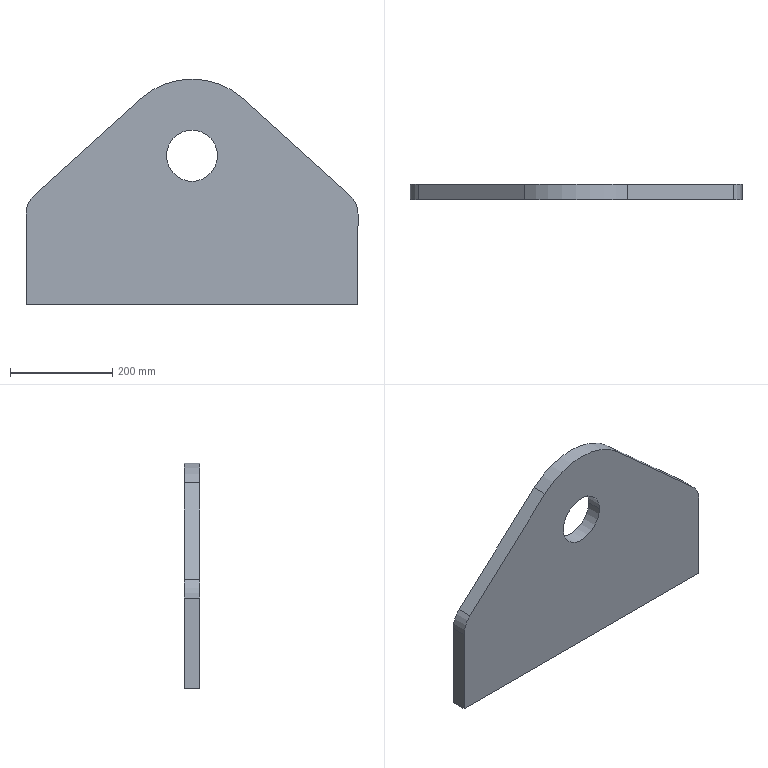Component | SolidWorks | Support1-1 | 1 solid | 12 faces | box 650 x 30 x 442 mm | volume 6416148 mm3 | plane 7 | cylinder 5 | commonest cylinder face diameters 100 x4 300 x1 | material Plain Carbon Steel
STEP:
#1=COLOUR_RGB('',0.7922,0.8196,0.9333);
#2=FILL_AREA_STYLE_COLOUR('',#1);
#3=FILL_AREA_STYLE('',(#2));
#4=SURFACE_STYLE_FILL_AREA(#3);
#5=SURFACE_SIDE_STYLE('',(#4));
#6=SURFACE_STYLE_USAGE(.BOTH.,#5);
#7=PRESENTATION_STYLE_ASSIGNMENT((#6));
#8=CARTESIAN_POINT('',(47.267,41.982,72.956));
#9=VERTEX_POINT('',#8);
#10=CARTESIAN_POINT('',(51.204,41.982,72.956));
#11=VERTEX_POINT('',#10);
#12=CARTESIAN_POINT('',(49.235,41.982,72.956));
#13=DIRECTION('',(0.,1.,0.));
#14=DIRECTION('',(1.,0.,0.));
#15=AXIS2_PLACEMENT_3D('',#12,#13,#14);
#16=CIRCLE('',#15,1.969);
#17=EDGE_CURVE('',#9,#11,#16,.T.);
#18=ORIENTED_EDGE('',*,*,#17,.F.);
#19=CARTESIAN_POINT('',(47.267,43.163,72.956));
#20=VERTEX_POINT('',#19);
#21=CARTESIAN_POINT('',(47.267,41.982,72.956));
#22=DIRECTION('',(0.,1.,0.));
#23=VECTOR('',#22,39.37);
#24=LINE('',#21,#23);
#25=EDGE_CURVE('',#9,#20,#24,.T.);
#26=ORIENTED_EDGE('',*,*,#25,.T.);
#27=CARTESIAN_POINT('',(51.204,43.163,72.956));
#28=VERTEX_POINT('',#27);
#29=CARTESIAN_POINT('',(49.235,43.163,72.956));
#30=DIRECTION('',(0.,1.,0.));
#31=DIRECTION('',(1.,0.,0.));
#32=AXIS2_PLACEMENT_3D('',#29,#30,#31);
#33=CIRCLE('',#32,1.969);
#34=EDGE_CURVE('',#20,#28,#33,.T.);
#35=ORIENTED_EDGE('',*,*,#34,.T.);
#36=CARTESIAN_POINT('',(51.204,41.982,72.956));
#37=DIRECTION('',(0.,1.,0.));
#38=VECTOR('',#37,39.37);
#39=LINE('',#36,#38);
#40=EDGE_CURVE('',#11,#28,#39,.T.);
#41=ORIENTED_EDGE('',*,*,#40,.F.);
#42=EDGE_LOOP('',(#18,#26,#35,#41));
#43=FACE_OUTER_BOUND('',#42,.T.);
#44=CARTESIAN_POINT('',(49.235,41.982,72.956));
#45=DIRECTION('',(0.,1.,0.));
#46=DIRECTION('',(1.,0.,0.));
#47=AXIS2_PLACEMENT_3D('',#44,#45,#46);
#48=CYLINDRICAL_SURFACE('',#47,1.969);
#49=ADVANCED_FACE('',(#43),#48,.F.);
#50=CARTESIAN_POINT('',(36.44,43.163,61.46));
#51=VERTEX_POINT('',#50);
#52=CARTESIAN_POINT('',(36.44,43.163,68.461));
#53=VERTEX_POINT('',#52);
#54=CARTESIAN_POINT('',(36.44,43.163,61.46));
#55=DIRECTION('',(0.,-0.,1.));
#56=VECTOR('',#55,39.37);
#57=LINE('',#54,#56);
#58=EDGE_CURVE('',#51,#53,#57,.T.);
#59=ORIENTED_EDGE('',*,*,#58,.F.);
#60=CARTESIAN_POINT('',(36.44,41.982,61.46));
#61=VERTEX_POINT('',#60);
#62=CARTESIAN_POINT('',(36.44,41.982,61.46));
#63=DIRECTION('',(0.,1.,0.));
#64=VECTOR('',#63,39.37);
#65=LINE('',#62,#64);
#66=EDGE_CURVE('',#61,#51,#65,.T.);
#67=ORIENTED_EDGE('',*,*,#66,.F.);
#68=CARTESIAN_POINT('',(36.44,41.982,68.461));
#69=VERTEX_POINT('',#68);
#70=CARTESIAN_POINT('',(36.44,41.982,61.46));
#71=DIRECTION('',(0.,-0.,1.));
#72=VECTOR('',#71,39.37);
#73=LINE('',#70,#72);
#74=EDGE_CURVE('',#61,#69,#73,.T.);
#75=ORIENTED_EDGE('',*,*,#74,.T.);
#76=CARTESIAN_POINT('',(36.44,41.982,68.461));
#77=DIRECTION('',(0.,1.,0.));
#78=VECTOR('',#77,39.37);
#79=LINE('',#76,#78);
#80=EDGE_CURVE('',#69,#53,#79,.T.);
#81=ORIENTED_EDGE('',*,*,#80,.T.);
#82=EDGE_LOOP('',(#59,#67,#75,#81));
#83=FACE_OUTER_BOUND('',#82,.T.);
#84=CARTESIAN_POINT('',(36.44,41.982,61.46));
#85=DIRECTION('',(-1.,0.,0.));
#86=DIRECTION('',(0.,1.,0.));
#87=AXIS2_PLACEMENT_3D('',#84,#85,#86);
#88=PLANE('',#87);
#89=ADVANCED_FACE('',(#83),#88,.T.);
#90=CARTESIAN_POINT('',(62.031,43.163,61.46));
#91=VERTEX_POINT('',#90);
#92=CARTESIAN_POINT('',(36.44,43.163,61.46));
#93=DIRECTION('',(-1.,0.,0.));
#94=VECTOR('',#93,39.37);
#95=LINE('',#92,#94);
#96=EDGE_CURVE('',#91,#51,#95,.T.);
#97=ORIENTED_EDGE('',*,*,#96,.F.);
#98=CARTESIAN_POINT('',(62.031,41.982,61.46));
#99=VERTEX_POINT('',#98);
#100=CARTESIAN_POINT('',(62.031,41.982,61.46));
#101=DIRECTION('',(0.,1.,0.));
#102=VECTOR('',#101,39.37);
#103=LINE('',#100,#102);
#104=EDGE_CURVE('',#99,#91,#103,.T.);
#105=ORIENTED_EDGE('',*,*,#104,.F.);
#106=CARTESIAN_POINT('',(36.44,41.982,61.46));
#107=DIRECTION('',(-1.,0.,0.));
#108=VECTOR('',#107,39.37);
#109=LINE('',#106,#108);
#110=EDGE_CURVE('',#99,#61,#109,.T.);
#111=ORIENTED_EDGE('',*,*,#110,.T.);
#112=ORIENTED_EDGE('',*,*,#66,.T.);
#113=EDGE_LOOP('',(#97,#105,#111,#112));
#114=FACE_OUTER_BOUND('',#113,.T.);
#115=CARTESIAN_POINT('',(36.44,41.982,61.46));
#116=DIRECTION('',(0.,0.,-1.));
#117=DIRECTION('',(0.,1.,0.));
#118=AXIS2_PLACEMENT_3D('',#115,#116,#117);
#119=PLANE('',#118);
#120=ADVANCED_FACE('',(#114),#119,.T.);
#121=CARTESIAN_POINT('',(62.031,43.163,68.461));
#122=VERTEX_POINT('',#121);
#123=CARTESIAN_POINT('',(62.031,43.163,61.46));
#124=DIRECTION('',(-0.,0.,-1.));
#125=VECTOR('',#124,39.37);
#126=LINE('',#123,#125);
#127=EDGE_CURVE('',#122,#91,#126,.T.);
#128=ORIENTED_EDGE('',*,*,#127,.F.);
#129=CARTESIAN_POINT('',(62.031,41.982,68.461));
#130=VERTEX_POINT('',#129);
#131=CARTESIAN_POINT('',(62.031,41.982,68.461));
#132=DIRECTION('',(0.,1.,0.));
#133=VECTOR('',#132,39.37);
#134=LINE('',#131,#133);
#135=EDGE_CURVE('',#130,#122,#134,.T.);
#136=ORIENTED_EDGE('',*,*,#135,.F.);
#137=CARTESIAN_POINT('',(62.031,41.982,61.46));
#138=DIRECTION('',(-0.,0.,-1.));
#139=VECTOR('',#138,39.37);
#140=LINE('',#137,#139);
#141=EDGE_CURVE('',#130,#99,#140,.T.);
#142=ORIENTED_EDGE('',*,*,#141,.T.);
#143=ORIENTED_EDGE('',*,*,#104,.T.);
#144=EDGE_LOOP('',(#128,#136,#142,#143));
#145=FACE_OUTER_BOUND('',#144,.T.);
#146=CARTESIAN_POINT('',(62.031,41.982,61.46));
#147=DIRECTION('',(1.,0.,-0.));
#148=DIRECTION('',(-0.,0.,-1.));
#149=AXIS2_PLACEMENT_3D('',#146,#147,#148);
#150=PLANE('',#149);
#151=ADVANCED_FACE('',(#145),#150,.T.);
#152=CARTESIAN_POINT('',(61.384,43.163,69.92));
#153=VERTEX_POINT('',#152);
#154=CARTESIAN_POINT('',(60.062,43.163,68.461));
#155=DIRECTION('',(0.,1.,0.));
#156=DIRECTION('',(1.,0.,0.));
#157=AXIS2_PLACEMENT_3D('',#154,#155,#156);
#158=CIRCLE('',#157,1.969);
#159=EDGE_CURVE('',#153,#122,#158,.T.);
#160=ORIENTED_EDGE('',*,*,#159,.F.);
#161=CARTESIAN_POINT('',(61.384,41.982,69.92));
#162=VERTEX_POINT('',#161);
#163=CARTESIAN_POINT('',(61.384,41.982,69.92));
#164=DIRECTION('',(0.,1.,0.));
#165=VECTOR('',#164,39.37);
#166=LINE('',#163,#165);
#167=EDGE_CURVE('',#162,#153,#166,.T.);
#168=ORIENTED_EDGE('',*,*,#167,.F.);
#169=CARTESIAN_POINT('',(60.062,41.982,68.461));
#170=DIRECTION('',(0.,1.,0.));
#171=DIRECTION('',(1.,0.,0.));
#172=AXIS2_PLACEMENT_3D('',#169,#170,#171);
#173=CIRCLE('',#172,1.969);
#174=EDGE_CURVE('',#162,#130,#173,.T.);
#175=ORIENTED_EDGE('',*,*,#174,.T.);
#176=ORIENTED_EDGE('',*,*,#135,.T.);
#177=EDGE_LOOP('',(#160,#168,#175,#176));
#178=FACE_OUTER_BOUND('',#177,.T.);
#179=CARTESIAN_POINT('',(60.062,41.982,68.461));
#180=DIRECTION('',(0.,1.,0.));
#181=DIRECTION('',(1.,0.,0.));
#182=AXIS2_PLACEMENT_3D('',#179,#180,#181);
#183=CYLINDRICAL_SURFACE('',#182,1.969);
#184=ADVANCED_FACE('',(#178),#183,.T.);
#185=CARTESIAN_POINT('',(53.2,43.163,77.333));
#186=VERTEX_POINT('',#185);
#187=CARTESIAN_POINT('',(61.384,43.163,69.92));
#188=DIRECTION('',(0.7411,0.,-0.6713));
#189=VECTOR('',#188,39.37);
#190=LINE('',#187,#189);
#191=EDGE_CURVE('',#186,#153,#190,.T.);
#192=ORIENTED_EDGE('',*,*,#191,.F.);
#193=CARTESIAN_POINT('',(53.2,41.982,77.333));
#194=VERTEX_POINT('',#193);
#195=CARTESIAN_POINT('',(53.2,41.982,77.333));
#196=DIRECTION('',(0.,1.,0.));
#197=VECTOR('',#196,39.37);
#198=LINE('',#195,#197);
#199=EDGE_CURVE('',#194,#186,#198,.T.);
#200=ORIENTED_EDGE('',*,*,#199,.F.);
#201=CARTESIAN_POINT('',(61.384,41.982,69.92));
#202=DIRECTION('',(0.7411,0.,-0.6713));
#203=VECTOR('',#202,39.37);
#204=LINE('',#201,#203);
#205=EDGE_CURVE('',#194,#162,#204,.T.);
#206=ORIENTED_EDGE('',*,*,#205,.T.);
#207=ORIENTED_EDGE('',*,*,#167,.T.);
#208=EDGE_LOOP('',(#192,#200,#206,#207));
#209=FACE_OUTER_BOUND('',#208,.T.);
#210=CARTESIAN_POINT('',(61.384,41.982,69.92));
#211=DIRECTION('',(0.6713,-0.,0.7411));
#212=DIRECTION('',(0.7411,0.,-0.6713));
#213=AXIS2_PLACEMENT_3D('',#210,#211,#212);
#214=PLANE('',#213);
#215=ADVANCED_FACE('',(#209),#214,.T.);
#216=CARTESIAN_POINT('',(45.271,43.163,77.333));
#217=VERTEX_POINT('',#216);
#218=CARTESIAN_POINT('',(49.235,43.163,72.956));
#219=DIRECTION('',(0.,1.,0.));
#220=DIRECTION('',(1.,0.,0.));
#221=AXIS2_PLACEMENT_3D('',#218,#219,#220);
#222=CIRCLE('',#221,5.906);
#223=EDGE_CURVE('',#217,#186,#222,.T.);
#224=ORIENTED_EDGE('',*,*,#223,.F.);
#225=CARTESIAN_POINT('',(45.271,41.982,77.333));
#226=VERTEX_POINT('',#225);
#227=CARTESIAN_POINT('',(45.271,41.982,77.333));
#228=DIRECTION('',(0.,1.,0.));
#229=VECTOR('',#228,39.37);
#230=LINE('',#227,#229);
#231=EDGE_CURVE('',#226,#217,#230,.T.);
#232=ORIENTED_EDGE('',*,*,#231,.F.);
#233=CARTESIAN_POINT('',(49.235,41.982,72.956));
#234=DIRECTION('',(0.,1.,0.));
#235=DIRECTION('',(1.,0.,0.));
#236=AXIS2_PLACEMENT_3D('',#233,#234,#235);
#237=CIRCLE('',#236,5.906);
#238=EDGE_CURVE('',#226,#194,#237,.T.);
#239=ORIENTED_EDGE('',*,*,#238,.T.);
#240=ORIENTED_EDGE('',*,*,#199,.T.);
#241=EDGE_LOOP('',(#224,#232,#239,#240));
#242=FACE_OUTER_BOUND('',#241,.T.);
#243=CARTESIAN_POINT('',(49.235,41.982,72.956));
#244=DIRECTION('',(0.,1.,0.));
#245=DIRECTION('',(1.,0.,0.));
#246=AXIS2_PLACEMENT_3D('',#243,#244,#245);
#247=CYLINDRICAL_SURFACE('',#246,5.906);
#248=ADVANCED_FACE('',(#242),#247,.T.);
#249=CARTESIAN_POINT('',(37.087,43.163,69.92));
#250=VERTEX_POINT('',#249);
#251=CARTESIAN_POINT('',(37.087,43.163,69.92));
#252=DIRECTION('',(0.7411,-0.,0.6713));
#253=VECTOR('',#252,39.37);
#254=LINE('',#251,#253);
#255=EDGE_CURVE('',#250,#217,#254,.T.);
#256=ORIENTED_EDGE('',*,*,#255,.F.);
#257=CARTESIAN_POINT('',(37.087,41.982,69.92));
#258=VERTEX_POINT('',#257);
#259=CARTESIAN_POINT('',(37.087,41.982,69.92));
#260=DIRECTION('',(0.,1.,0.));
#261=VECTOR('',#260,39.37);
#262=LINE('',#259,#261);
#263=EDGE_CURVE('',#258,#250,#262,.T.);
#264=ORIENTED_EDGE('',*,*,#263,.F.);
#265=CARTESIAN_POINT('',(37.087,41.982,69.92));
#266=DIRECTION('',(0.7411,-0.,0.6713));
#267=VECTOR('',#266,39.37);
#268=LINE('',#265,#267);
#269=EDGE_CURVE('',#258,#226,#268,.T.);
#270=ORIENTED_EDGE('',*,*,#269,.T.);
#271=ORIENTED_EDGE('',*,*,#231,.T.);
#272=EDGE_LOOP('',(#256,#264,#270,#271));
#273=FACE_OUTER_BOUND('',#272,.T.);
#274=CARTESIAN_POINT('',(37.087,41.982,69.92));
#275=DIRECTION('',(-0.6713,-0.,0.7411));
#276=DIRECTION('',(0.7411,-0.,0.6713));
#277=AXIS2_PLACEMENT_3D('',#274,#275,#276);
#278=PLANE('',#277);
#279=ADVANCED_FACE('',(#273),#278,.T.);
#280=CARTESIAN_POINT('',(38.409,43.163,68.461));
#281=DIRECTION('',(0.,1.,0.));
#282=DIRECTION('',(-1.,0.,0.));
#283=AXIS2_PLACEMENT_3D('',#280,#281,#282);
#284=CIRCLE('',#283,1.969);
#285=EDGE_CURVE('',#53,#250,#284,.T.);
#286=ORIENTED_EDGE('',*,*,#285,.F.);
#287=ORIENTED_EDGE('',*,*,#80,.F.);
#288=CARTESIAN_POINT('',(38.409,41.982,68.461));
#289=DIRECTION('',(0.,1.,0.));
#290=DIRECTION('',(-1.,0.,0.));
#291=AXIS2_PLACEMENT_3D('',#288,#289,#290);
#292=CIRCLE('',#291,1.969);
#293=EDGE_CURVE('',#69,#258,#292,.T.);
#294=ORIENTED_EDGE('',*,*,#293,.T.);
#295=ORIENTED_EDGE('',*,*,#263,.T.);
#296=EDGE_LOOP('',(#286,#287,#294,#295));
#297=FACE_OUTER_BOUND('',#296,.T.);
#298=CARTESIAN_POINT('',(38.409,41.982,68.461));
#299=DIRECTION('',(0.,1.,0.));
#300=DIRECTION('',(1.,0.,0.));
#301=AXIS2_PLACEMENT_3D('',#298,#299,#300);
#302=CYLINDRICAL_SURFACE('',#301,1.969);
#303=ADVANCED_FACE('',(#297),#302,.T.);
#304=CARTESIAN_POINT('',(49.235,41.982,72.956));
#305=DIRECTION('',(0.,1.,0.));
#306=DIRECTION('',(1.,0.,0.));
#307=AXIS2_PLACEMENT_3D('',#304,#305,#306);
#308=CIRCLE('',#307,1.969);
#309=EDGE_CURVE('',#11,#9,#308,.T.);
#310=ORIENTED_EDGE('',*,*,#309,.T.);
#311=ORIENTED_EDGE('',*,*,#17,.T.);
#312=EDGE_LOOP('',(#310,#311));
#313=FACE_BOUND('',#312,.T.);
#314=ORIENTED_EDGE('',*,*,#74,.F.);
#315=ORIENTED_EDGE('',*,*,#110,.F.);
#316=ORIENTED_EDGE('',*,*,#141,.F.);
#317=ORIENTED_EDGE('',*,*,#174,.F.);
#318=ORIENTED_EDGE('',*,*,#205,.F.);
#319=ORIENTED_EDGE('',*,*,#238,.F.);
#320=ORIENTED_EDGE('',*,*,#269,.F.);
#321=ORIENTED_EDGE('',*,*,#293,.F.);
#322=EDGE_LOOP('',(#314,#315,#316,#317,#318,#319,#320,#321));
#323=FACE_OUTER_BOUND('',#322,.T.);
#324=CARTESIAN_POINT('',(38.409,41.982,68.461));
#325=DIRECTION('',(0.,-1.,-0.));
#326=DIRECTION('',(-1.,0.,0.));
#327=AXIS2_PLACEMENT_3D('',#324,#325,#326);
#328=PLANE('',#327);
#329=ADVANCED_FACE('',(#313,#323),#328,.T.);
#330=CARTESIAN_POINT('',(49.235,43.163,72.956));
#331=DIRECTION('',(0.,1.,0.));
#332=DIRECTION('',(1.,0.,0.));
#333=AXIS2_PLACEMENT_3D('',#330,#331,#332);
#334=CIRCLE('',#333,1.969);
#335=EDGE_CURVE('',#28,#20,#334,.T.);
#336=ORIENTED_EDGE('',*,*,#335,.F.);
#337=ORIENTED_EDGE('',*,*,#34,.F.);
#338=EDGE_LOOP('',(#336,#337));
#339=FACE_BOUND('',#338,.T.);
#340=ORIENTED_EDGE('',*,*,#58,.T.);
#341=ORIENTED_EDGE('',*,*,#285,.T.);
#342=ORIENTED_EDGE('',*,*,#255,.T.);
#343=ORIENTED_EDGE('',*,*,#223,.T.);
#344=ORIENTED_EDGE('',*,*,#191,.T.);
#345=ORIENTED_EDGE('',*,*,#159,.T.);
#346=ORIENTED_EDGE('',*,*,#127,.T.);
#347=ORIENTED_EDGE('',*,*,#96,.T.);
#348=EDGE_LOOP('',(#340,#341,#342,#343,#344,#345,#346,#347));
#349=FACE_OUTER_BOUND('',#348,.T.);
#350=CARTESIAN_POINT('',(38.409,43.163,68.461));
#351=DIRECTION('',(0.,-1.,-0.));
#352=DIRECTION('',(-1.,0.,0.));
#353=AXIS2_PLACEMENT_3D('',#350,#351,#352);
#354=PLANE('',#353);
#355=ADVANCED_FACE('',(#339,#349),#354,.F.);
#356=ORIENTED_EDGE('',*,*,#25,.F.);
#357=ORIENTED_EDGE('',*,*,#309,.F.);
#358=ORIENTED_EDGE('',*,*,#40,.T.);
#359=ORIENTED_EDGE('',*,*,#335,.T.);
#360=EDGE_LOOP('',(#356,#357,#358,#359));
#361=FACE_OUTER_BOUND('',#360,.T.);
#362=CARTESIAN_POINT('',(49.235,41.982,72.956));
#363=DIRECTION('',(0.,1.,0.));
#364=DIRECTION('',(1.,0.,0.));
#365=AXIS2_PLACEMENT_3D('',#362,#363,#364);
#366=CYLINDRICAL_SURFACE('',#365,1.969);
#367=ADVANCED_FACE('',(#361),#366,.F.);
#368=CLOSED_SHELL('',(#49,#89,#120,#151,#184,#215,#248,#279,#303,#329,#355,#367));
#369=MANIFOLD_SOLID_BREP('',#368);
#370=STYLED_ITEM('',(#7),#369);
#371=(LENGTH_UNIT()NAMED_UNIT(*)SI_UNIT($,.METRE.));
#372=LENGTH_MEASURE_WITH_UNIT(LENGTH_MEASURE(0.0254),#371);
#373=DIMENSIONAL_EXPONENTS(1.,0.,0.,0.,0.,0.,0.);
#374=(CONVERSION_BASED_UNIT('',#372)LENGTH_UNIT()NAMED_UNIT(#373));
#375=UNCERTAINTY_MEASURE_WITH_UNIT(LENGTH_MEASURE(0.00001),#374,'','');
#376=(NAMED_UNIT(*)PLANE_ANGLE_UNIT()SI_UNIT($,.RADIAN.));
#377=(NAMED_UNIT(*)SI_UNIT($,.STERADIAN.)SOLID_ANGLE_UNIT());
#378=(GEOMETRIC_REPRESENTATION_CONTEXT(3)GLOBAL_UNCERTAINTY_ASSIGNED_CONTEXT((#375))GLOBAL_UNIT_ASSIGNED_CONTEXT((#374,#376,#377))REPRESENTATION_CONTEXT('',''));
#379=MECHANICAL_DESIGN_GEOMETRIC_PRESENTATION_REPRESENTATION('',(#370),#378);
#380=CARTESIAN_POINT('',(0.,0.,0.));
#381=DIRECTION('',(0.,0.,1.));
#382=DIRECTION('',(1.,0.,0.));
#383=AXIS2_PLACEMENT_3D('',#380,#381,#382);
#384=(LENGTH_UNIT()NAMED_UNIT(*)SI_UNIT($,.METRE.));
#385=LENGTH_MEASURE_WITH_UNIT(LENGTH_MEASURE(0.0254),#384);
#386=DIMENSIONAL_EXPONENTS(1.,0.,0.,0.,0.,0.,0.);
#387=(CONVERSION_BASED_UNIT('',#385)LENGTH_UNIT()NAMED_UNIT(#386));
#388=UNCERTAINTY_MEASURE_WITH_UNIT(LENGTH_MEASURE(0.00001),#387,'','');
#389=(NAMED_UNIT(*)PLANE_ANGLE_UNIT()SI_UNIT($,.RADIAN.));
#390=(NAMED_UNIT(*)SI_UNIT($,.STERADIAN.)SOLID_ANGLE_UNIT());
#391=(GEOMETRIC_REPRESENTATION_CONTEXT(3)GLOBAL_UNCERTAINTY_ASSIGNED_CONTEXT((#388))GLOBAL_UNIT_ASSIGNED_CONTEXT((#387,#389,#390))REPRESENTATION_CONTEXT('',''));
#392=ADVANCED_BREP_SHAPE_REPRESENTATION('',(#369,#383),#391);
#393=PRESENTATION_LAYER_ASSIGNMENT('','',(#370));